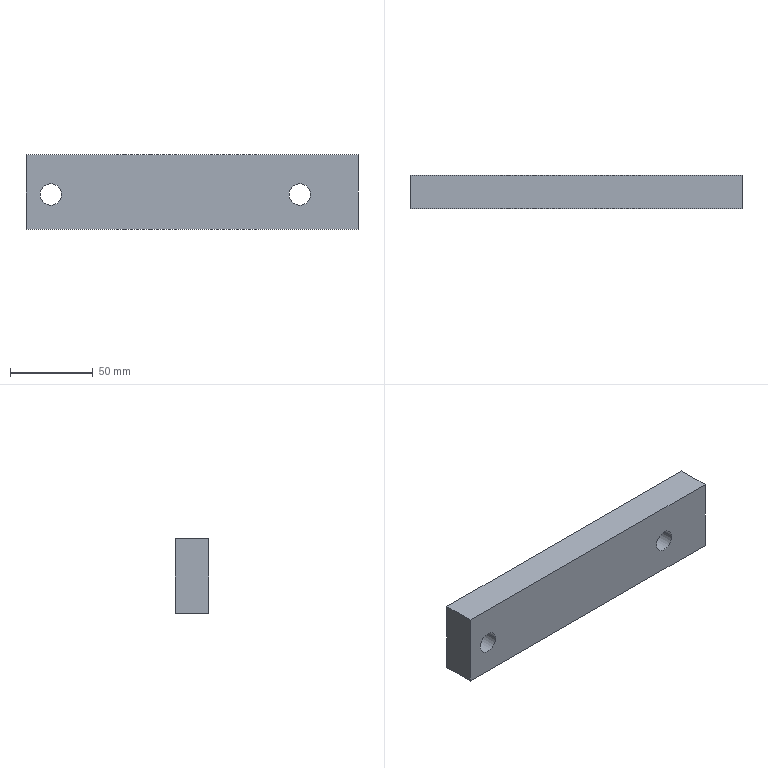Component | SolidWorks | NewTypeCurveBenderReinforcement-1 | 1 solid | 10 faces | box 200 x 20 x 45 mm | volume 174691 mm3 | plane 6 | cylinder 4 | commonest cylinder face diameters 13 x4
build123d program:
from build123d import *

# Parameters (mm, degrees)
SKETCH1_W           = 45
SKETCH1_H           = 20
BOSS_EXTRUDE1_DEPTH = 200
SKETCH2_R           = 6.5
CUT_EXTRUDE1_DEPTH  = 414


with BuildPart() as part:
    # Sketch1 → Boss-Extrude1 (new body)
    with BuildSketch(Plane.XY):
        with Locations((22.5, 10)):
            Rectangle(SKETCH1_W, SKETCH1_H)
    extrude(amount=BOSS_EXTRUDE1_DEPTH)

    # Sketch2 → Cut-Extrude1 (cut)
    with BuildSketch(Plane.XZ):
        with Locations(Location((24, 15, 0), (0, 0, 270))):
            Circle(SKETCH2_R)
        with Locations(Location((24, 165, 0), (0, 0, 270))):
            Circle(SKETCH2_R)
    extrude(amount=-CUT_EXTRUDE1_DEPTH, mode=Mode.SUBTRACT)


solid = part.part

# Placed as in the assembly
solid = solid.moved(Location((-90, 96, 318.11), (0, 90, 0)))
STEP:
#1=COLOUR_RGB('',0.7922,0.8196,0.9333);
#2=FILL_AREA_STYLE_COLOUR('',#1);
#3=FILL_AREA_STYLE('',(#2));
#4=SURFACE_STYLE_FILL_AREA(#3);
#5=SURFACE_SIDE_STYLE('',(#4));
#6=SURFACE_STYLE_USAGE(.BOTH.,#5);
#7=PRESENTATION_STYLE_ASSIGNMENT((#6));
#8=CARTESIAN_POINT('',(-2.697,4.567,11.579));
#9=VERTEX_POINT('',#8);
#10=CARTESIAN_POINT('',(-3.209,4.567,11.579));
#11=VERTEX_POINT('',#10);
#12=CARTESIAN_POINT('',(-2.953,4.567,11.579));
#13=DIRECTION('',(0.,-1.,-0.));
#14=DIRECTION('',(-1.,0.,0.));
#15=AXIS2_PLACEMENT_3D('',#12,#13,#14);
#16=CIRCLE('',#15,0.2559);
#17=EDGE_CURVE('',#9,#11,#16,.T.);
#18=ORIENTED_EDGE('',*,*,#17,.F.);
#19=CARTESIAN_POINT('',(-2.697,3.78,11.579));
#20=VERTEX_POINT('',#19);
#21=CARTESIAN_POINT('',(-2.697,20.079,11.579));
#22=DIRECTION('',(0.,-1.,-0.));
#23=VECTOR('',#22,39.37);
#24=LINE('',#21,#23);
#25=EDGE_CURVE('',#9,#20,#24,.T.);
#26=ORIENTED_EDGE('',*,*,#25,.T.);
#27=CARTESIAN_POINT('',(-3.209,3.78,11.579));
#28=VERTEX_POINT('',#27);
#29=CARTESIAN_POINT('',(-2.953,3.78,11.579));
#30=DIRECTION('',(0.,-1.,-0.));
#31=DIRECTION('',(-1.,0.,0.));
#32=AXIS2_PLACEMENT_3D('',#29,#30,#31);
#33=CIRCLE('',#32,0.2559);
#34=EDGE_CURVE('',#20,#28,#33,.T.);
#35=ORIENTED_EDGE('',*,*,#34,.T.);
#36=CARTESIAN_POINT('',(-3.209,20.079,11.579));
#37=DIRECTION('',(0.,-1.,-0.));
#38=VECTOR('',#37,39.37);
#39=LINE('',#36,#38);
#40=EDGE_CURVE('',#11,#28,#39,.T.);
#41=ORIENTED_EDGE('',*,*,#40,.F.);
#42=EDGE_LOOP('',(#18,#26,#35,#41));
#43=FACE_OUTER_BOUND('',#42,.T.);
#44=CARTESIAN_POINT('',(-2.953,20.079,11.579));
#45=DIRECTION('',(0.,-1.,-0.));
#46=DIRECTION('',(-1.,0.,0.));
#47=AXIS2_PLACEMENT_3D('',#44,#45,#46);
#48=CYLINDRICAL_SURFACE('',#47,0.2559);
#49=ADVANCED_FACE('',(#43),#48,.F.);
#50=CARTESIAN_POINT('',(3.209,4.567,11.579));
#51=VERTEX_POINT('',#50);
#52=CARTESIAN_POINT('',(2.697,4.567,11.579));
#53=VERTEX_POINT('',#52);
#54=CARTESIAN_POINT('',(2.953,4.567,11.579));
#55=DIRECTION('',(0.,-1.,-0.));
#56=DIRECTION('',(-1.,0.,0.));
#57=AXIS2_PLACEMENT_3D('',#54,#55,#56);
#58=CIRCLE('',#57,0.2559);
#59=EDGE_CURVE('',#51,#53,#58,.T.);
#60=ORIENTED_EDGE('',*,*,#59,.F.);
#61=CARTESIAN_POINT('',(3.209,3.78,11.579));
#62=VERTEX_POINT('',#61);
#63=CARTESIAN_POINT('',(3.209,20.079,11.579));
#64=DIRECTION('',(0.,-1.,-0.));
#65=VECTOR('',#64,39.37);
#66=LINE('',#63,#65);
#67=EDGE_CURVE('',#51,#62,#66,.T.);
#68=ORIENTED_EDGE('',*,*,#67,.T.);
#69=CARTESIAN_POINT('',(2.697,3.78,11.579));
#70=VERTEX_POINT('',#69);
#71=CARTESIAN_POINT('',(2.953,3.78,11.579));
#72=DIRECTION('',(0.,-1.,-0.));
#73=DIRECTION('',(-1.,0.,0.));
#74=AXIS2_PLACEMENT_3D('',#71,#72,#73);
#75=CIRCLE('',#74,0.2559);
#76=EDGE_CURVE('',#62,#70,#75,.T.);
#77=ORIENTED_EDGE('',*,*,#76,.T.);
#78=CARTESIAN_POINT('',(2.697,20.079,11.579));
#79=DIRECTION('',(0.,-1.,-0.));
#80=VECTOR('',#79,39.37);
#81=LINE('',#78,#80);
#82=EDGE_CURVE('',#53,#70,#81,.T.);
#83=ORIENTED_EDGE('',*,*,#82,.F.);
#84=EDGE_LOOP('',(#60,#68,#77,#83));
#85=FACE_OUTER_BOUND('',#84,.T.);
#86=CARTESIAN_POINT('',(2.953,20.079,11.579));
#87=DIRECTION('',(0.,-1.,-0.));
#88=DIRECTION('',(-1.,0.,0.));
#89=AXIS2_PLACEMENT_3D('',#86,#87,#88);
#90=CYLINDRICAL_SURFACE('',#89,0.2559);
#91=ADVANCED_FACE('',(#85),#90,.F.);
#92=CARTESIAN_POINT('',(-3.543,4.567,12.524));
#93=VERTEX_POINT('',#92);
#94=CARTESIAN_POINT('',(-3.543,3.78,12.524));
#95=VERTEX_POINT('',#94);
#96=CARTESIAN_POINT('',(-3.543,3.78,12.524));
#97=DIRECTION('',(0.,-1.,-0.));
#98=VECTOR('',#97,39.37);
#99=LINE('',#96,#98);
#100=EDGE_CURVE('',#93,#95,#99,.T.);
#101=ORIENTED_EDGE('',*,*,#100,.T.);
#102=CARTESIAN_POINT('',(4.331,3.78,12.524));
#103=VERTEX_POINT('',#102);
#104=CARTESIAN_POINT('',(4.331,3.78,12.524));
#105=DIRECTION('',(-1.,-0.,0.));
#106=VECTOR('',#105,39.37);
#107=LINE('',#104,#106);
#108=EDGE_CURVE('',#103,#95,#107,.T.);
#109=ORIENTED_EDGE('',*,*,#108,.F.);
#110=CARTESIAN_POINT('',(4.331,4.567,12.524));
#111=VERTEX_POINT('',#110);
#112=CARTESIAN_POINT('',(4.331,3.78,12.524));
#113=DIRECTION('',(0.,-1.,-0.));
#114=VECTOR('',#113,39.37);
#115=LINE('',#112,#114);
#116=EDGE_CURVE('',#111,#103,#115,.T.);
#117=ORIENTED_EDGE('',*,*,#116,.F.);
#118=CARTESIAN_POINT('',(4.331,4.567,12.524));
#119=DIRECTION('',(-1.,-0.,0.));
#120=VECTOR('',#119,39.37);
#121=LINE('',#118,#120);
#122=EDGE_CURVE('',#111,#93,#121,.T.);
#123=ORIENTED_EDGE('',*,*,#122,.T.);
#124=EDGE_LOOP('',(#101,#109,#117,#123));
#125=FACE_OUTER_BOUND('',#124,.T.);
#126=CARTESIAN_POINT('',(4.331,3.78,12.524));
#127=DIRECTION('',(-0.,0.,-1.));
#128=DIRECTION('',(-1.,-0.,0.));
#129=AXIS2_PLACEMENT_3D('',#126,#127,#128);
#130=PLANE('',#129);
#131=ADVANCED_FACE('',(#125),#130,.F.);
#132=CARTESIAN_POINT('',(-2.953,3.78,11.579));
#133=DIRECTION('',(0.,-1.,-0.));
#134=DIRECTION('',(-1.,0.,0.));
#135=AXIS2_PLACEMENT_3D('',#132,#133,#134);
#136=CIRCLE('',#135,0.2559);
#137=EDGE_CURVE('',#28,#20,#136,.T.);
#138=ORIENTED_EDGE('',*,*,#137,.F.);
#139=ORIENTED_EDGE('',*,*,#34,.F.);
#140=EDGE_LOOP('',(#138,#139));
#141=FACE_BOUND('',#140,.T.);
#142=CARTESIAN_POINT('',(2.953,3.78,11.579));
#143=DIRECTION('',(0.,-1.,-0.));
#144=DIRECTION('',(-1.,0.,0.));
#145=AXIS2_PLACEMENT_3D('',#142,#143,#144);
#146=CIRCLE('',#145,0.2559);
#147=EDGE_CURVE('',#70,#62,#146,.T.);
#148=ORIENTED_EDGE('',*,*,#147,.F.);
#149=ORIENTED_EDGE('',*,*,#76,.F.);
#150=EDGE_LOOP('',(#148,#149));
#151=FACE_BOUND('',#150,.T.);
#152=CARTESIAN_POINT('',(-3.543,3.78,10.752));
#153=VERTEX_POINT('',#152);
#154=CARTESIAN_POINT('',(-3.543,3.78,12.524));
#155=DIRECTION('',(-0.,0.,-1.));
#156=VECTOR('',#155,39.37);
#157=LINE('',#154,#156);
#158=EDGE_CURVE('',#95,#153,#157,.T.);
#159=ORIENTED_EDGE('',*,*,#158,.T.);
#160=CARTESIAN_POINT('',(4.331,3.78,10.752));
#161=VERTEX_POINT('',#160);
#162=CARTESIAN_POINT('',(4.331,3.78,10.752));
#163=DIRECTION('',(-1.,-0.,0.));
#164=VECTOR('',#163,39.37);
#165=LINE('',#162,#164);
#166=EDGE_CURVE('',#161,#153,#165,.T.);
#167=ORIENTED_EDGE('',*,*,#166,.F.);
#168=CARTESIAN_POINT('',(4.331,3.78,12.524));
#169=DIRECTION('',(-0.,0.,-1.));
#170=VECTOR('',#169,39.37);
#171=LINE('',#168,#170);
#172=EDGE_CURVE('',#103,#161,#171,.T.);
#173=ORIENTED_EDGE('',*,*,#172,.F.);
#174=ORIENTED_EDGE('',*,*,#108,.T.);
#175=EDGE_LOOP('',(#159,#167,#173,#174));
#176=FACE_OUTER_BOUND('',#175,.T.);
#177=CARTESIAN_POINT('',(4.331,3.78,12.524));
#178=DIRECTION('',(-0.,1.,0.));
#179=DIRECTION('',(1.,0.,-0.));
#180=AXIS2_PLACEMENT_3D('',#177,#178,#179);
#181=PLANE('',#180);
#182=ADVANCED_FACE('',(#141,#151,#176),#181,.F.);
#183=CARTESIAN_POINT('',(-3.543,4.567,10.752));
#184=VERTEX_POINT('',#183);
#185=CARTESIAN_POINT('',(-3.543,3.78,10.752));
#186=DIRECTION('',(-0.,1.,0.));
#187=VECTOR('',#186,39.37);
#188=LINE('',#185,#187);
#189=EDGE_CURVE('',#153,#184,#188,.T.);
#190=ORIENTED_EDGE('',*,*,#189,.T.);
#191=CARTESIAN_POINT('',(4.331,4.567,10.752));
#192=VERTEX_POINT('',#191);
#193=CARTESIAN_POINT('',(4.331,4.567,10.752));
#194=DIRECTION('',(-1.,-0.,0.));
#195=VECTOR('',#194,39.37);
#196=LINE('',#193,#195);
#197=EDGE_CURVE('',#192,#184,#196,.T.);
#198=ORIENTED_EDGE('',*,*,#197,.F.);
#199=CARTESIAN_POINT('',(4.331,3.78,10.752));
#200=DIRECTION('',(-0.,1.,0.));
#201=VECTOR('',#200,39.37);
#202=LINE('',#199,#201);
#203=EDGE_CURVE('',#161,#192,#202,.T.);
#204=ORIENTED_EDGE('',*,*,#203,.F.);
#205=ORIENTED_EDGE('',*,*,#166,.T.);
#206=EDGE_LOOP('',(#190,#198,#204,#205));
#207=FACE_OUTER_BOUND('',#206,.T.);
#208=CARTESIAN_POINT('',(4.331,3.78,10.752));
#209=DIRECTION('',(0.,-0.,1.));
#210=DIRECTION('',(1.,0.,-0.));
#211=AXIS2_PLACEMENT_3D('',#208,#209,#210);
#212=PLANE('',#211);
#213=ADVANCED_FACE('',(#207),#212,.F.);
#214=CARTESIAN_POINT('',(-2.953,4.567,11.579));
#215=DIRECTION('',(0.,-1.,-0.));
#216=DIRECTION('',(-1.,0.,0.));
#217=AXIS2_PLACEMENT_3D('',#214,#215,#216);
#218=CIRCLE('',#217,0.2559);
#219=EDGE_CURVE('',#11,#9,#218,.T.);
#220=ORIENTED_EDGE('',*,*,#219,.T.);
#221=ORIENTED_EDGE('',*,*,#17,.T.);
#222=EDGE_LOOP('',(#220,#221));
#223=FACE_BOUND('',#222,.T.);
#224=CARTESIAN_POINT('',(2.953,4.567,11.579));
#225=DIRECTION('',(0.,-1.,-0.));
#226=DIRECTION('',(-1.,0.,0.));
#227=AXIS2_PLACEMENT_3D('',#224,#225,#226);
#228=CIRCLE('',#227,0.2559);
#229=EDGE_CURVE('',#53,#51,#228,.T.);
#230=ORIENTED_EDGE('',*,*,#229,.T.);
#231=ORIENTED_EDGE('',*,*,#59,.T.);
#232=EDGE_LOOP('',(#230,#231));
#233=FACE_BOUND('',#232,.T.);
#234=CARTESIAN_POINT('',(-3.543,4.567,12.524));
#235=DIRECTION('',(0.,-0.,1.));
#236=VECTOR('',#235,39.37);
#237=LINE('',#234,#236);
#238=EDGE_CURVE('',#184,#93,#237,.T.);
#239=ORIENTED_EDGE('',*,*,#238,.T.);
#240=ORIENTED_EDGE('',*,*,#122,.F.);
#241=CARTESIAN_POINT('',(4.331,4.567,12.524));
#242=DIRECTION('',(0.,-0.,1.));
#243=VECTOR('',#242,39.37);
#244=LINE('',#241,#243);
#245=EDGE_CURVE('',#192,#111,#244,.T.);
#246=ORIENTED_EDGE('',*,*,#245,.F.);
#247=ORIENTED_EDGE('',*,*,#197,.T.);
#248=EDGE_LOOP('',(#239,#240,#246,#247));
#249=FACE_OUTER_BOUND('',#248,.T.);
#250=CARTESIAN_POINT('',(4.331,4.567,12.524));
#251=DIRECTION('',(0.,-1.,-0.));
#252=DIRECTION('',(-1.,-0.,0.));
#253=AXIS2_PLACEMENT_3D('',#250,#251,#252);
#254=PLANE('',#253);
#255=ADVANCED_FACE('',(#223,#233,#249),#254,.F.);
#256=ORIENTED_EDGE('',*,*,#116,.T.);
#257=ORIENTED_EDGE('',*,*,#172,.T.);
#258=ORIENTED_EDGE('',*,*,#203,.T.);
#259=ORIENTED_EDGE('',*,*,#245,.T.);
#260=EDGE_LOOP('',(#256,#257,#258,#259));
#261=FACE_OUTER_BOUND('',#260,.T.);
#262=CARTESIAN_POINT('',(4.331,3.78,12.524));
#263=DIRECTION('',(-1.,-0.,0.));
#264=DIRECTION('',(0.,-0.,1.));
#265=AXIS2_PLACEMENT_3D('',#262,#263,#264);
#266=PLANE('',#265);
#267=ADVANCED_FACE('',(#261),#266,.F.);
#268=ORIENTED_EDGE('',*,*,#100,.F.);
#269=ORIENTED_EDGE('',*,*,#238,.F.);
#270=ORIENTED_EDGE('',*,*,#189,.F.);
#271=ORIENTED_EDGE('',*,*,#158,.F.);
#272=EDGE_LOOP('',(#268,#269,#270,#271));
#273=FACE_OUTER_BOUND('',#272,.T.);
#274=CARTESIAN_POINT('',(-3.543,3.78,12.524));
#275=DIRECTION('',(-1.,-0.,0.));
#276=DIRECTION('',(0.,-0.,1.));
#277=AXIS2_PLACEMENT_3D('',#274,#275,#276);
#278=PLANE('',#277);
#279=ADVANCED_FACE('',(#273),#278,.T.);
#280=ORIENTED_EDGE('',*,*,#67,.F.);
#281=ORIENTED_EDGE('',*,*,#229,.F.);
#282=ORIENTED_EDGE('',*,*,#82,.T.);
#283=ORIENTED_EDGE('',*,*,#147,.T.);
#284=EDGE_LOOP('',(#280,#281,#282,#283));
#285=FACE_OUTER_BOUND('',#284,.T.);
#286=CARTESIAN_POINT('',(2.953,20.079,11.579));
#287=DIRECTION('',(0.,-1.,-0.));
#288=DIRECTION('',(-1.,0.,0.));
#289=AXIS2_PLACEMENT_3D('',#286,#287,#288);
#290=CYLINDRICAL_SURFACE('',#289,0.2559);
#291=ADVANCED_FACE('',(#285),#290,.F.);
#292=ORIENTED_EDGE('',*,*,#25,.F.);
#293=ORIENTED_EDGE('',*,*,#219,.F.);
#294=ORIENTED_EDGE('',*,*,#40,.T.);
#295=ORIENTED_EDGE('',*,*,#137,.T.);
#296=EDGE_LOOP('',(#292,#293,#294,#295));
#297=FACE_OUTER_BOUND('',#296,.T.);
#298=CARTESIAN_POINT('',(-2.953,20.079,11.579));
#299=DIRECTION('',(0.,-1.,-0.));
#300=DIRECTION('',(-1.,0.,0.));
#301=AXIS2_PLACEMENT_3D('',#298,#299,#300);
#302=CYLINDRICAL_SURFACE('',#301,0.2559);
#303=ADVANCED_FACE('',(#297),#302,.F.);
#304=CLOSED_SHELL('',(#49,#91,#131,#182,#213,#255,#267,#279,#291,#303));
#305=MANIFOLD_SOLID_BREP('',#304);
#306=STYLED_ITEM('',(#7),#305);
#307=PRESENTATION_LAYER_ASSIGNMENT('','',(#306));
#308=(LENGTH_UNIT()NAMED_UNIT(*)SI_UNIT($,.METRE.));
#309=LENGTH_MEASURE_WITH_UNIT(LENGTH_MEASURE(0.0254),#308);
#310=DIMENSIONAL_EXPONENTS(1.,0.,0.,0.,0.,0.,0.);
#311=(CONVERSION_BASED_UNIT('',#309)LENGTH_UNIT()NAMED_UNIT(#310));
#312=UNCERTAINTY_MEASURE_WITH_UNIT(LENGTH_MEASURE(0.00001),#311,'','');
#313=(NAMED_UNIT(*)PLANE_ANGLE_UNIT()SI_UNIT($,.RADIAN.));
#314=(NAMED_UNIT(*)SI_UNIT($,.STERADIAN.)SOLID_ANGLE_UNIT());
#315=(GEOMETRIC_REPRESENTATION_CONTEXT(3)GLOBAL_UNCERTAINTY_ASSIGNED_CONTEXT((#312))GLOBAL_UNIT_ASSIGNED_CONTEXT((#311,#313,#314))REPRESENTATION_CONTEXT('',''));
#316=MECHANICAL_DESIGN_GEOMETRIC_PRESENTATION_REPRESENTATION('',(#306),#315);
#317=CARTESIAN_POINT('',(0.,0.,0.));
#318=DIRECTION('',(0.,0.,1.));
#319=DIRECTION('',(1.,0.,0.));
#320=AXIS2_PLACEMENT_3D('',#317,#318,#319);
#321=(LENGTH_UNIT()NAMED_UNIT(*)SI_UNIT($,.METRE.));
#322=LENGTH_MEASURE_WITH_UNIT(LENGTH_MEASURE(0.0254),#321);
#323=DIMENSIONAL_EXPONENTS(1.,0.,0.,0.,0.,0.,0.);
#324=(CONVERSION_BASED_UNIT('',#322)LENGTH_UNIT()NAMED_UNIT(#323));
#325=UNCERTAINTY_MEASURE_WITH_UNIT(LENGTH_MEASURE(0.00001),#324,'','');
#326=(NAMED_UNIT(*)PLANE_ANGLE_UNIT()SI_UNIT($,.RADIAN.));
#327=(NAMED_UNIT(*)SI_UNIT($,.STERADIAN.)SOLID_ANGLE_UNIT());
#328=(GEOMETRIC_REPRESENTATION_CONTEXT(3)GLOBAL_UNCERTAINTY_ASSIGNED_CONTEXT((#325))GLOBAL_UNIT_ASSIGNED_CONTEXT((#324,#326,#327))REPRESENTATION_CONTEXT('',''));
#329=ADVANCED_BREP_SHAPE_REPRESENTATION('',(#305,#320),#328);